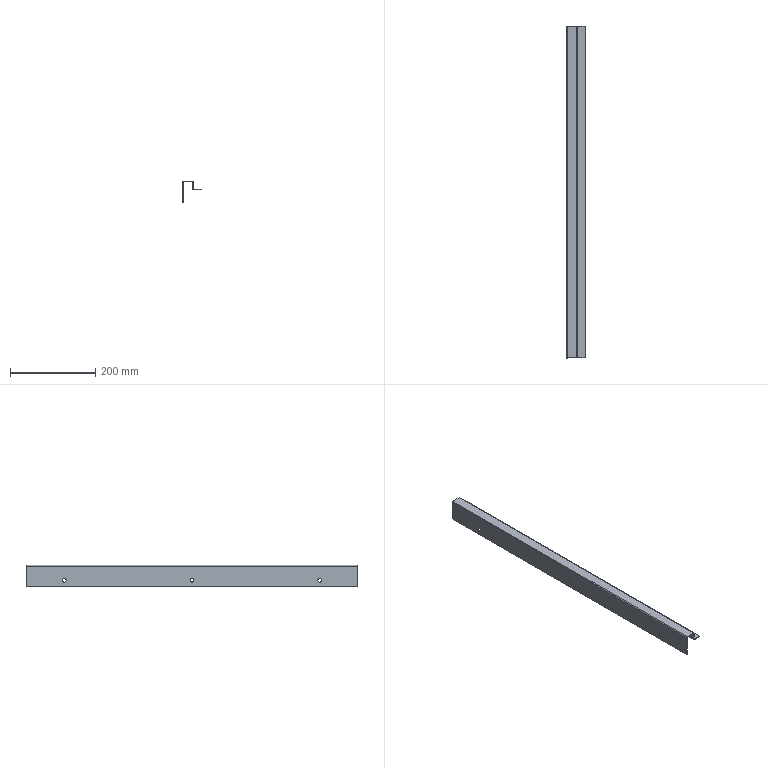Component | SolidWorks | Column-1 | 1 solid | 36 faces | box 43.5 x 780 x 50 mm | volume 127718 mm3 | plane 24 | cylinder 12 | commonest cylinder face diameters 9 x6 3.2 x3 0.2 x3
STEP:
#1=CARTESIAN_POINT('',(-13.498,9.896,34.139));
#2=VERTEX_POINT('',#1);
#3=CARTESIAN_POINT('',(-13.498,9.896,34.494));
#4=VERTEX_POINT('',#3);
#5=CARTESIAN_POINT('',(-13.498,9.896,34.316));
#6=DIRECTION('',(-1.,-0.,0.));
#7=DIRECTION('',(0.,0.,1.));
#8=AXIS2_PLACEMENT_3D('',#5,#6,#7);
#9=CIRCLE('',#8,0.1772);
#10=EDGE_CURVE('',#2,#4,#9,.T.);
#11=ORIENTED_EDGE('',*,*,#10,.T.);
#12=CARTESIAN_POINT('',(-13.439,9.896,34.494));
#13=VERTEX_POINT('',#12);
#14=CARTESIAN_POINT('',(-13.833,9.896,34.494));
#15=DIRECTION('',(1.,0.,-0.));
#16=VECTOR('',#15,39.37);
#17=LINE('',#14,#16);
#18=EDGE_CURVE('',#4,#13,#17,.T.);
#19=ORIENTED_EDGE('',*,*,#18,.T.);
#20=CARTESIAN_POINT('',(-13.439,9.896,34.139));
#21=VERTEX_POINT('',#20);
#22=CARTESIAN_POINT('',(-13.439,9.896,34.316));
#23=DIRECTION('',(1.,0.,-0.));
#24=DIRECTION('',(0.,0.,-1.));
#25=AXIS2_PLACEMENT_3D('',#22,#23,#24);
#26=CIRCLE('',#25,0.1772);
#27=EDGE_CURVE('',#13,#21,#26,.T.);
#28=ORIENTED_EDGE('',*,*,#27,.T.);
#29=CARTESIAN_POINT('',(-13.833,9.896,34.139));
#30=DIRECTION('',(1.,0.,-0.));
#31=VECTOR('',#30,39.37);
#32=LINE('',#29,#31);
#33=EDGE_CURVE('',#2,#21,#32,.T.);
#34=ORIENTED_EDGE('',*,*,#33,.F.);
#35=EDGE_LOOP('',(#11,#19,#28,#34));
#36=FACE_OUTER_BOUND('',#35,.T.);
#37=CARTESIAN_POINT('',(-13.833,9.896,34.316));
#38=DIRECTION('',(1.,0.,-0.));
#39=DIRECTION('',(0.,0.,-1.));
#40=AXIS2_PLACEMENT_3D('',#37,#38,#39);
#41=CYLINDRICAL_SURFACE('',#40,0.1772);
#42=ADVANCED_FACE('',(#36),#41,.F.);
#43=CARTESIAN_POINT('',(-13.498,-13.726,34.139));
#44=VERTEX_POINT('',#43);
#45=CARTESIAN_POINT('',(-13.498,-13.726,34.494));
#46=VERTEX_POINT('',#45);
#47=CARTESIAN_POINT('',(-13.498,-13.726,34.316));
#48=DIRECTION('',(-1.,-0.,0.));
#49=DIRECTION('',(0.,0.,1.));
#50=AXIS2_PLACEMENT_3D('',#47,#48,#49);
#51=CIRCLE('',#50,0.1772);
#52=EDGE_CURVE('',#44,#46,#51,.T.);
#53=ORIENTED_EDGE('',*,*,#52,.T.);
#54=CARTESIAN_POINT('',(-13.439,-13.726,34.494));
#55=VERTEX_POINT('',#54);
#56=CARTESIAN_POINT('',(-13.833,-13.726,34.494));
#57=DIRECTION('',(1.,0.,-0.));
#58=VECTOR('',#57,39.37);
#59=LINE('',#56,#58);
#60=EDGE_CURVE('',#46,#55,#59,.T.);
#61=ORIENTED_EDGE('',*,*,#60,.T.);
#62=CARTESIAN_POINT('',(-13.439,-13.726,34.139));
#63=VERTEX_POINT('',#62);
#64=CARTESIAN_POINT('',(-13.439,-13.726,34.316));
#65=DIRECTION('',(1.,0.,-0.));
#66=DIRECTION('',(0.,0.,-1.));
#67=AXIS2_PLACEMENT_3D('',#64,#65,#66);
#68=CIRCLE('',#67,0.1772);
#69=EDGE_CURVE('',#55,#63,#68,.T.);
#70=ORIENTED_EDGE('',*,*,#69,.T.);
#71=CARTESIAN_POINT('',(-13.833,-13.726,34.139));
#72=DIRECTION('',(1.,0.,-0.));
#73=VECTOR('',#72,39.37);
#74=LINE('',#71,#73);
#75=EDGE_CURVE('',#44,#63,#74,.T.);
#76=ORIENTED_EDGE('',*,*,#75,.F.);
#77=EDGE_LOOP('',(#53,#61,#70,#76));
#78=FACE_OUTER_BOUND('',#77,.T.);
#79=CARTESIAN_POINT('',(-13.833,-13.726,34.316));
#80=DIRECTION('',(1.,0.,-0.));
#81=DIRECTION('',(0.,0.,-1.));
#82=AXIS2_PLACEMENT_3D('',#79,#80,#81);
#83=CYLINDRICAL_SURFACE('',#82,0.1772);
#84=ADVANCED_FACE('',(#78),#83,.F.);
#85=CARTESIAN_POINT('',(-13.498,-1.915,34.139));
#86=VERTEX_POINT('',#85);
#87=CARTESIAN_POINT('',(-13.498,-1.915,34.494));
#88=VERTEX_POINT('',#87);
#89=CARTESIAN_POINT('',(-13.498,-1.915,34.316));
#90=DIRECTION('',(-1.,-0.,0.));
#91=DIRECTION('',(0.,0.,1.));
#92=AXIS2_PLACEMENT_3D('',#89,#90,#91);
#93=CIRCLE('',#92,0.1772);
#94=EDGE_CURVE('',#86,#88,#93,.T.);
#95=ORIENTED_EDGE('',*,*,#94,.T.);
#96=CARTESIAN_POINT('',(-13.439,-1.915,34.494));
#97=VERTEX_POINT('',#96);
#98=CARTESIAN_POINT('',(-13.833,-1.915,34.494));
#99=DIRECTION('',(1.,0.,-0.));
#100=VECTOR('',#99,39.37);
#101=LINE('',#98,#100);
#102=EDGE_CURVE('',#88,#97,#101,.T.);
#103=ORIENTED_EDGE('',*,*,#102,.T.);
#104=CARTESIAN_POINT('',(-13.439,-1.915,34.139));
#105=VERTEX_POINT('',#104);
#106=CARTESIAN_POINT('',(-13.439,-1.915,34.316));
#107=DIRECTION('',(1.,0.,-0.));
#108=DIRECTION('',(0.,0.,-1.));
#109=AXIS2_PLACEMENT_3D('',#106,#107,#108);
#110=CIRCLE('',#109,0.1772);
#111=EDGE_CURVE('',#97,#105,#110,.T.);
#112=ORIENTED_EDGE('',*,*,#111,.T.);
#113=CARTESIAN_POINT('',(-13.833,-1.915,34.139));
#114=DIRECTION('',(1.,0.,-0.));
#115=VECTOR('',#114,39.37);
#116=LINE('',#113,#115);
#117=EDGE_CURVE('',#86,#105,#116,.T.);
#118=ORIENTED_EDGE('',*,*,#117,.F.);
#119=EDGE_LOOP('',(#95,#103,#112,#118));
#120=FACE_OUTER_BOUND('',#119,.T.);
#121=CARTESIAN_POINT('',(-13.833,-1.915,34.316));
#122=DIRECTION('',(1.,0.,-0.));
#123=DIRECTION('',(0.,0.,-1.));
#124=AXIS2_PLACEMENT_3D('',#121,#122,#123);
#125=CYLINDRICAL_SURFACE('',#124,0.1772);
#126=ADVANCED_FACE('',(#120),#125,.F.);
#127=CARTESIAN_POINT('',(-12.514,13.44,35.631));
#128=VERTEX_POINT('',#127);
#129=CARTESIAN_POINT('',(-12.514,13.44,34.97));
#130=VERTEX_POINT('',#129);
#131=CARTESIAN_POINT('',(-12.514,13.44,34.907));
#132=DIRECTION('',(0.,0.,-1.));
#133=VECTOR('',#132,39.37);
#134=LINE('',#131,#133);
#135=EDGE_CURVE('',#128,#130,#134,.T.);
#136=ORIENTED_EDGE('',*,*,#135,.T.);
#137=CARTESIAN_POINT('',(-12.573,13.44,34.97));
#138=VERTEX_POINT('',#137);
#139=CARTESIAN_POINT('',(-12.514,13.44,34.97));
#140=DIRECTION('',(-1.,0.,0.));
#141=VECTOR('',#140,39.37);
#142=LINE('',#139,#141);
#143=EDGE_CURVE('',#130,#138,#142,.T.);
#144=ORIENTED_EDGE('',*,*,#143,.T.);
#145=CARTESIAN_POINT('',(-12.573,13.44,35.631));
#146=VERTEX_POINT('',#145);
#147=CARTESIAN_POINT('',(-12.573,13.44,35.694));
#148=DIRECTION('',(0.,0.,-1.));
#149=VECTOR('',#148,39.37);
#150=LINE('',#147,#149);
#151=EDGE_CURVE('',#146,#138,#150,.T.);
#152=ORIENTED_EDGE('',*,*,#151,.F.);
#153=CARTESIAN_POINT('',(-12.514,13.44,35.631));
#154=DIRECTION('',(1.,0.,0.));
#155=VECTOR('',#154,39.37);
#156=LINE('',#153,#155);
#157=EDGE_CURVE('',#146,#128,#156,.T.);
#158=ORIENTED_EDGE('',*,*,#157,.T.);
#159=EDGE_LOOP('',(#136,#144,#152,#158));
#160=FACE_OUTER_BOUND('',#159,.T.);
#161=CARTESIAN_POINT('',(-12.514,13.44,34.907));
#162=DIRECTION('',(-0.,1.,-0.));
#163=DIRECTION('',(-1.,-0.,0.));
#164=AXIS2_PLACEMENT_3D('',#161,#162,#163);
#165=PLANE('',#164);
#166=ADVANCED_FACE('',(#160),#165,.T.);
#167=CARTESIAN_POINT('',(-12.514,-17.269,34.97));
#168=VERTEX_POINT('',#167);
#169=CARTESIAN_POINT('',(-12.514,-17.269,35.631));
#170=VERTEX_POINT('',#169);
#171=CARTESIAN_POINT('',(-12.514,-17.269,35.635));
#172=DIRECTION('',(-0.,-0.,1.));
#173=VECTOR('',#172,39.37);
#174=LINE('',#171,#173);
#175=EDGE_CURVE('',#168,#170,#174,.T.);
#176=ORIENTED_EDGE('',*,*,#175,.F.);
#177=CARTESIAN_POINT('',(-12.514,13.44,34.97));
#178=DIRECTION('',(0.,-1.,0.));
#179=VECTOR('',#178,39.37);
#180=LINE('',#177,#179);
#181=EDGE_CURVE('',#130,#168,#180,.T.);
#182=ORIENTED_EDGE('',*,*,#181,.F.);
#183=ORIENTED_EDGE('',*,*,#135,.F.);
#184=CARTESIAN_POINT('',(-12.514,-1.915,35.631));
#185=DIRECTION('',(0.,-1.,0.));
#186=VECTOR('',#185,39.37);
#187=LINE('',#184,#186);
#188=EDGE_CURVE('',#128,#170,#187,.T.);
#189=ORIENTED_EDGE('',*,*,#188,.T.);
#190=EDGE_LOOP('',(#176,#182,#183,#189));
#191=FACE_OUTER_BOUND('',#190,.T.);
#192=CARTESIAN_POINT('',(-12.514,-1.915,35.694));
#193=DIRECTION('',(1.,0.,0.));
#194=DIRECTION('',(0.,0.,-1.));
#195=AXIS2_PLACEMENT_3D('',#192,#193,#194);
#196=PLANE('',#195);
#197=ADVANCED_FACE('',(#191),#196,.T.);
#198=CARTESIAN_POINT('',(-12.573,-17.269,34.97));
#199=VERTEX_POINT('',#198);
#200=CARTESIAN_POINT('',(-12.573,13.44,34.97));
#201=DIRECTION('',(0.,-1.,0.));
#202=VECTOR('',#201,39.37);
#203=LINE('',#200,#202);
#204=EDGE_CURVE('',#138,#199,#203,.T.);
#205=ORIENTED_EDGE('',*,*,#204,.T.);
#206=CARTESIAN_POINT('',(-12.573,-17.269,35.631));
#207=VERTEX_POINT('',#206);
#208=CARTESIAN_POINT('',(-12.573,-17.269,35.694));
#209=DIRECTION('',(-0.,-0.,1.));
#210=VECTOR('',#209,39.37);
#211=LINE('',#208,#210);
#212=EDGE_CURVE('',#199,#207,#211,.T.);
#213=ORIENTED_EDGE('',*,*,#212,.T.);
#214=CARTESIAN_POINT('',(-12.573,13.44,35.631));
#215=DIRECTION('',(0.,-1.,0.));
#216=VECTOR('',#215,39.37);
#217=LINE('',#214,#216);
#218=EDGE_CURVE('',#146,#207,#217,.T.);
#219=ORIENTED_EDGE('',*,*,#218,.F.);
#220=ORIENTED_EDGE('',*,*,#151,.T.);
#221=EDGE_LOOP('',(#205,#213,#219,#220));
#222=FACE_OUTER_BOUND('',#221,.T.);
#223=CARTESIAN_POINT('',(-12.573,-1.915,35.694));
#224=DIRECTION('',(1.,0.,0.));
#225=DIRECTION('',(0.,0.,-1.));
#226=AXIS2_PLACEMENT_3D('',#223,#224,#225);
#227=PLANE('',#226);
#228=ADVANCED_FACE('',(#222),#227,.F.);
#229=CARTESIAN_POINT('',(-12.577,-17.269,35.635));
#230=VERTEX_POINT('',#229);
#231=CARTESIAN_POINT('',(-12.577,13.44,35.635));
#232=VERTEX_POINT('',#231);
#233=CARTESIAN_POINT('',(-12.577,-17.269,35.635));
#234=DIRECTION('',(0.,1.,0.));
#235=VECTOR('',#234,39.37);
#236=LINE('',#233,#235);
#237=EDGE_CURVE('',#230,#232,#236,.T.);
#238=ORIENTED_EDGE('',*,*,#237,.F.);
#239=CARTESIAN_POINT('',(-13.435,-17.269,35.635));
#240=VERTEX_POINT('',#239);
#241=CARTESIAN_POINT('',(-13.498,-17.269,35.635));
#242=DIRECTION('',(1.,0.,0.));
#243=VECTOR('',#242,39.37);
#244=LINE('',#241,#243);
#245=EDGE_CURVE('',#240,#230,#244,.T.);
#246=ORIENTED_EDGE('',*,*,#245,.F.);
#247=CARTESIAN_POINT('',(-13.435,13.44,35.635));
#248=VERTEX_POINT('',#247);
#249=CARTESIAN_POINT('',(-13.435,13.44,35.635));
#250=DIRECTION('',(0.,-1.,0.));
#251=VECTOR('',#250,39.37);
#252=LINE('',#249,#251);
#253=EDGE_CURVE('',#248,#240,#252,.T.);
#254=ORIENTED_EDGE('',*,*,#253,.F.);
#255=CARTESIAN_POINT('',(-13.498,13.44,35.635));
#256=DIRECTION('',(-1.,0.,0.));
#257=VECTOR('',#256,39.37);
#258=LINE('',#255,#257);
#259=EDGE_CURVE('',#232,#248,#258,.T.);
#260=ORIENTED_EDGE('',*,*,#259,.F.);
#261=EDGE_LOOP('',(#238,#246,#254,#260));
#262=FACE_OUTER_BOUND('',#261,.T.);
#263=CARTESIAN_POINT('',(-13.006,-1.915,35.635));
#264=DIRECTION('',(0.,0.,1.));
#265=DIRECTION('',(1.,0.,0.));
#266=AXIS2_PLACEMENT_3D('',#263,#264,#265);
#267=PLANE('',#266);
#268=ADVANCED_FACE('',(#262),#267,.F.);
#269=CARTESIAN_POINT('',(-13.435,-17.269,35.694));
#270=VERTEX_POINT('',#269);
#271=CARTESIAN_POINT('',(-12.577,-17.269,35.694));
#272=VERTEX_POINT('',#271);
#273=CARTESIAN_POINT('',(-13.498,-17.269,35.694));
#274=DIRECTION('',(1.,0.,0.));
#275=VECTOR('',#274,39.37);
#276=LINE('',#273,#275);
#277=EDGE_CURVE('',#270,#272,#276,.T.);
#278=ORIENTED_EDGE('',*,*,#277,.T.);
#279=CARTESIAN_POINT('',(-12.577,13.44,35.694));
#280=VERTEX_POINT('',#279);
#281=CARTESIAN_POINT('',(-12.577,-17.269,35.694));
#282=DIRECTION('',(0.,1.,0.));
#283=VECTOR('',#282,39.37);
#284=LINE('',#281,#283);
#285=EDGE_CURVE('',#272,#280,#284,.T.);
#286=ORIENTED_EDGE('',*,*,#285,.T.);
#287=CARTESIAN_POINT('',(-13.435,13.44,35.694));
#288=VERTEX_POINT('',#287);
#289=CARTESIAN_POINT('',(-13.498,13.44,35.694));
#290=DIRECTION('',(-1.,0.,0.));
#291=VECTOR('',#290,39.37);
#292=LINE('',#289,#291);
#293=EDGE_CURVE('',#280,#288,#292,.T.);
#294=ORIENTED_EDGE('',*,*,#293,.T.);
#295=CARTESIAN_POINT('',(-13.435,13.44,35.694));
#296=DIRECTION('',(0.,-1.,0.));
#297=VECTOR('',#296,39.37);
#298=LINE('',#295,#297);
#299=EDGE_CURVE('',#288,#270,#298,.T.);
#300=ORIENTED_EDGE('',*,*,#299,.T.);
#301=EDGE_LOOP('',(#278,#286,#294,#300));
#302=FACE_OUTER_BOUND('',#301,.T.);
#303=CARTESIAN_POINT('',(-13.006,-1.915,35.694));
#304=DIRECTION('',(0.,0.,1.));
#305=DIRECTION('',(1.,0.,0.));
#306=AXIS2_PLACEMENT_3D('',#303,#304,#305);
#307=PLANE('',#306);
#308=ADVANCED_FACE('',(#302),#307,.T.);
#309=ORIENTED_EDGE('',*,*,#245,.T.);
#310=CARTESIAN_POINT('',(-12.577,-17.269,35.635));
#311=DIRECTION('',(0.,0.,1.));
#312=VECTOR('',#311,39.37);
#313=LINE('',#310,#312);
#314=EDGE_CURVE('',#230,#272,#313,.T.);
#315=ORIENTED_EDGE('',*,*,#314,.T.);
#316=ORIENTED_EDGE('',*,*,#277,.F.);
#317=CARTESIAN_POINT('',(-13.435,-17.269,35.635));
#318=DIRECTION('',(-0.,0.,1.));
#319=VECTOR('',#318,39.37);
#320=LINE('',#317,#319);
#321=EDGE_CURVE('',#240,#270,#320,.T.);
#322=ORIENTED_EDGE('',*,*,#321,.F.);
#323=EDGE_LOOP('',(#309,#315,#316,#322));
#324=FACE_OUTER_BOUND('',#323,.T.);
#325=CARTESIAN_POINT('',(-13.498,-17.269,35.635));
#326=DIRECTION('',(0.,-1.,0.));
#327=DIRECTION('',(0.,0.,-1.));
#328=AXIS2_PLACEMENT_3D('',#325,#326,#327);
#329=PLANE('',#328);
#330=ADVANCED_FACE('',(#324),#329,.T.);
#331=CARTESIAN_POINT('',(-12.577,13.44,35.635));
#332=DIRECTION('',(0.,0.,1.));
#333=VECTOR('',#332,39.37);
#334=LINE('',#331,#333);
#335=EDGE_CURVE('',#232,#280,#334,.T.);
#336=ORIENTED_EDGE('',*,*,#335,.F.);
#337=ORIENTED_EDGE('',*,*,#259,.T.);
#338=CARTESIAN_POINT('',(-13.435,13.44,35.635));
#339=DIRECTION('',(-0.,0.,1.));
#340=VECTOR('',#339,39.37);
#341=LINE('',#338,#340);
#342=EDGE_CURVE('',#248,#288,#341,.T.);
#343=ORIENTED_EDGE('',*,*,#342,.T.);
#344=ORIENTED_EDGE('',*,*,#293,.F.);
#345=EDGE_LOOP('',(#336,#337,#343,#344));
#346=FACE_OUTER_BOUND('',#345,.T.);
#347=CARTESIAN_POINT('',(-13.498,13.44,35.635));
#348=DIRECTION('',(0.,1.,0.));
#349=DIRECTION('',(0.,0.,1.));
#350=AXIS2_PLACEMENT_3D('',#347,#348,#349);
#351=PLANE('',#350);
#352=ADVANCED_FACE('',(#346),#351,.T.);
#353=CARTESIAN_POINT('',(-13.439,-17.269,35.631));
#354=VERTEX_POINT('',#353);
#355=CARTESIAN_POINT('',(-13.498,-17.269,35.631));
#356=VERTEX_POINT('',#355);
#357=CARTESIAN_POINT('',(-13.498,-17.269,35.631));
#358=DIRECTION('',(-1.,-0.,0.));
#359=VECTOR('',#358,39.37);
#360=LINE('',#357,#359);
#361=EDGE_CURVE('',#354,#356,#360,.T.);
#362=ORIENTED_EDGE('',*,*,#361,.F.);
#363=CARTESIAN_POINT('',(-13.435,-17.269,35.631));
#364=DIRECTION('',(0.,-1.,0.));
#365=DIRECTION('',(-0.,0.,1.));
#366=AXIS2_PLACEMENT_3D('',#363,#364,#365);
#367=CIRCLE('',#366,0.003937);
#368=EDGE_CURVE('',#240,#354,#367,.T.);
#369=ORIENTED_EDGE('',*,*,#368,.F.);
#370=ORIENTED_EDGE('',*,*,#321,.T.);
#371=CARTESIAN_POINT('',(-13.435,-17.269,35.631));
#372=DIRECTION('',(0.,-1.,0.));
#373=DIRECTION('',(-0.,0.,1.));
#374=AXIS2_PLACEMENT_3D('',#371,#372,#373);
#375=CIRCLE('',#374,0.06299);
#376=EDGE_CURVE('',#270,#356,#375,.T.);
#377=ORIENTED_EDGE('',*,*,#376,.T.);
#378=EDGE_LOOP('',(#362,#369,#370,#377));
#379=FACE_OUTER_BOUND('',#378,.T.);
#380=CARTESIAN_POINT('',(-13.435,-17.269,35.631));
#381=DIRECTION('',(0.,-1.,0.));
#382=DIRECTION('',(0.,0.,-1.));
#383=AXIS2_PLACEMENT_3D('',#380,#381,#382);
#384=PLANE('',#383);
#385=ADVANCED_FACE('',(#379),#384,.T.);
#386=CARTESIAN_POINT('',(-13.439,13.44,35.631));
#387=VERTEX_POINT('',#386);
#388=CARTESIAN_POINT('',(-13.435,13.44,35.631));
#389=DIRECTION('',(0.,1.,0.));
#390=DIRECTION('',(0.,0.,1.));
#391=AXIS2_PLACEMENT_3D('',#388,#389,#390);
#392=CIRCLE('',#391,0.003937);
#393=EDGE_CURVE('',#387,#248,#392,.T.);
#394=ORIENTED_EDGE('',*,*,#393,.F.);
#395=CARTESIAN_POINT('',(-13.498,13.44,35.631));
#396=VERTEX_POINT('',#395);
#397=CARTESIAN_POINT('',(-13.439,13.44,35.631));
#398=DIRECTION('',(-1.,-0.,0.));
#399=VECTOR('',#398,39.37);
#400=LINE('',#397,#399);
#401=EDGE_CURVE('',#387,#396,#400,.T.);
#402=ORIENTED_EDGE('',*,*,#401,.T.);
#403=CARTESIAN_POINT('',(-13.435,13.44,35.631));
#404=DIRECTION('',(0.,1.,0.));
#405=DIRECTION('',(0.,0.,1.));
#406=AXIS2_PLACEMENT_3D('',#403,#404,#405);
#407=CIRCLE('',#406,0.06299);
#408=EDGE_CURVE('',#396,#288,#407,.T.);
#409=ORIENTED_EDGE('',*,*,#408,.T.);
#410=ORIENTED_EDGE('',*,*,#342,.F.);
#411=EDGE_LOOP('',(#394,#402,#409,#410));
#412=FACE_OUTER_BOUND('',#411,.T.);
#413=CARTESIAN_POINT('',(-13.435,13.44,35.631));
#414=DIRECTION('',(0.,-1.,0.));
#415=DIRECTION('',(0.,0.,-1.));
#416=AXIS2_PLACEMENT_3D('',#413,#414,#415);
#417=PLANE('',#416);
#418=ADVANCED_FACE('',(#412),#417,.F.);
#419=ORIENTED_EDGE('',*,*,#299,.F.);
#420=ORIENTED_EDGE('',*,*,#408,.F.);
#421=CARTESIAN_POINT('',(-13.498,-1.915,35.631));
#422=DIRECTION('',(-0.,1.,0.));
#423=VECTOR('',#422,39.37);
#424=LINE('',#421,#423);
#425=EDGE_CURVE('',#356,#396,#424,.T.);
#426=ORIENTED_EDGE('',*,*,#425,.F.);
#427=ORIENTED_EDGE('',*,*,#376,.F.);
#428=EDGE_LOOP('',(#419,#420,#426,#427));
#429=FACE_OUTER_BOUND('',#428,.T.);
#430=CARTESIAN_POINT('',(-13.435,13.44,35.631));
#431=DIRECTION('',(0.,1.,0.));
#432=DIRECTION('',(-1.,0.,0.));
#433=AXIS2_PLACEMENT_3D('',#430,#431,#432);
#434=CYLINDRICAL_SURFACE('',#433,0.06299);
#435=ADVANCED_FACE('',(#429),#434,.T.);
#436=ORIENTED_EDGE('',*,*,#253,.T.);
#437=ORIENTED_EDGE('',*,*,#368,.T.);
#438=CARTESIAN_POINT('',(-13.439,-17.269,35.631));
#439=DIRECTION('',(-0.,1.,0.));
#440=VECTOR('',#439,39.37);
#441=LINE('',#438,#440);
#442=EDGE_CURVE('',#354,#387,#441,.T.);
#443=ORIENTED_EDGE('',*,*,#442,.T.);
#444=ORIENTED_EDGE('',*,*,#393,.T.);
#445=EDGE_LOOP('',(#436,#437,#443,#444));
#446=FACE_OUTER_BOUND('',#445,.T.);
#447=CARTESIAN_POINT('',(-13.435,13.44,35.631));
#448=DIRECTION('',(0.,1.,0.));
#449=DIRECTION('',(-1.,0.,0.));
#450=AXIS2_PLACEMENT_3D('',#447,#448,#449);
#451=CYLINDRICAL_SURFACE('',#450,0.003937);
#452=ADVANCED_FACE('',(#446),#451,.F.);
#453=CARTESIAN_POINT('',(-13.498,13.44,33.726));
#454=VERTEX_POINT('',#453);
#455=CARTESIAN_POINT('',(-13.498,13.44,35.635));
#456=DIRECTION('',(0.,0.,1.));
#457=VECTOR('',#456,39.37);
#458=LINE('',#455,#457);
#459=EDGE_CURVE('',#454,#396,#458,.T.);
#460=ORIENTED_EDGE('',*,*,#459,.T.);
#461=ORIENTED_EDGE('',*,*,#401,.F.);
#462=CARTESIAN_POINT('',(-13.439,13.44,33.726));
#463=VERTEX_POINT('',#462);
#464=CARTESIAN_POINT('',(-13.439,13.44,35.694));
#465=DIRECTION('',(0.,0.,1.));
#466=VECTOR('',#465,39.37);
#467=LINE('',#464,#466);
#468=EDGE_CURVE('',#463,#387,#467,.T.);
#469=ORIENTED_EDGE('',*,*,#468,.F.);
#470=CARTESIAN_POINT('',(-13.498,13.44,33.726));
#471=DIRECTION('',(1.,0.,-0.));
#472=VECTOR('',#471,39.37);
#473=LINE('',#470,#472);
#474=EDGE_CURVE('',#454,#463,#473,.T.);
#475=ORIENTED_EDGE('',*,*,#474,.F.);
#476=EDGE_LOOP('',(#460,#461,#469,#475));
#477=FACE_OUTER_BOUND('',#476,.T.);
#478=CARTESIAN_POINT('',(-13.498,13.44,35.635));
#479=DIRECTION('',(-0.,1.,0.));
#480=DIRECTION('',(-1.,-0.,0.));
#481=AXIS2_PLACEMENT_3D('',#478,#479,#480);
#482=PLANE('',#481);
#483=ADVANCED_FACE('',(#477),#482,.T.);
#484=CARTESIAN_POINT('',(-13.439,-17.269,33.726));
#485=VERTEX_POINT('',#484);
#486=CARTESIAN_POINT('',(-13.439,-17.269,35.694));
#487=DIRECTION('',(-0.,0.,-1.));
#488=VECTOR('',#487,39.37);
#489=LINE('',#486,#488);
#490=EDGE_CURVE('',#354,#485,#489,.T.);
#491=ORIENTED_EDGE('',*,*,#490,.F.);
#492=ORIENTED_EDGE('',*,*,#361,.T.);
#493=CARTESIAN_POINT('',(-13.498,-17.269,33.726));
#494=VERTEX_POINT('',#493);
#495=CARTESIAN_POINT('',(-13.498,-17.269,33.726));
#496=DIRECTION('',(-0.,0.,-1.));
#497=VECTOR('',#496,39.37);
#498=LINE('',#495,#497);
#499=EDGE_CURVE('',#356,#494,#498,.T.);
#500=ORIENTED_EDGE('',*,*,#499,.T.);
#501=CARTESIAN_POINT('',(-13.498,-17.269,33.726));
#502=DIRECTION('',(1.,0.,-0.));
#503=VECTOR('',#502,39.37);
#504=LINE('',#501,#503);
#505=EDGE_CURVE('',#494,#485,#504,.T.);
#506=ORIENTED_EDGE('',*,*,#505,.T.);
#507=EDGE_LOOP('',(#491,#492,#500,#506));
#508=FACE_OUTER_BOUND('',#507,.T.);
#509=CARTESIAN_POINT('',(-13.498,-17.269,33.726));
#510=DIRECTION('',(0.,-1.,-0.));
#511=DIRECTION('',(1.,0.,0.));
#512=AXIS2_PLACEMENT_3D('',#509,#510,#511);
#513=PLANE('',#512);
#514=ADVANCED_FACE('',(#508),#513,.T.);
#515=ORIENTED_EDGE('',*,*,#52,.F.);
#516=CARTESIAN_POINT('',(-13.498,-13.726,34.316));
#517=DIRECTION('',(-1.,-0.,0.));
#518=DIRECTION('',(0.,0.,1.));
#519=AXIS2_PLACEMENT_3D('',#516,#517,#518);
#520=CIRCLE('',#519,0.1772);
#521=EDGE_CURVE('',#46,#44,#520,.T.);
#522=ORIENTED_EDGE('',*,*,#521,.F.);
#523=EDGE_LOOP('',(#515,#522));
#524=FACE_BOUND('',#523,.T.);
#525=ORIENTED_EDGE('',*,*,#94,.F.);
#526=CARTESIAN_POINT('',(-13.498,-1.915,34.316));
#527=DIRECTION('',(-1.,-0.,0.));
#528=DIRECTION('',(0.,0.,1.));
#529=AXIS2_PLACEMENT_3D('',#526,#527,#528);
#530=CIRCLE('',#529,0.1772);
#531=EDGE_CURVE('',#88,#86,#530,.T.);
#532=ORIENTED_EDGE('',*,*,#531,.F.);
#533=EDGE_LOOP('',(#525,#532));
#534=FACE_BOUND('',#533,.T.);
#535=ORIENTED_EDGE('',*,*,#499,.F.);
#536=ORIENTED_EDGE('',*,*,#425,.T.);
#537=ORIENTED_EDGE('',*,*,#459,.F.);
#538=CARTESIAN_POINT('',(-13.498,13.44,33.726));
#539=DIRECTION('',(-0.,1.,0.));
#540=VECTOR('',#539,39.37);
#541=LINE('',#538,#540);
#542=EDGE_CURVE('',#494,#454,#541,.T.);
#543=ORIENTED_EDGE('',*,*,#542,.F.);
#544=EDGE_LOOP('',(#535,#536,#537,#543));
#545=FACE_OUTER_BOUND('',#544,.T.);
#546=ORIENTED_EDGE('',*,*,#10,.F.);
#547=CARTESIAN_POINT('',(-13.498,9.896,34.316));
#548=DIRECTION('',(-1.,-0.,0.));
#549=DIRECTION('',(0.,0.,1.));
#550=AXIS2_PLACEMENT_3D('',#547,#548,#549);
#551=CIRCLE('',#550,0.1772);
#552=EDGE_CURVE('',#4,#2,#551,.T.);
#553=ORIENTED_EDGE('',*,*,#552,.F.);
#554=EDGE_LOOP('',(#546,#553));
#555=FACE_BOUND('',#554,.T.);
#556=CARTESIAN_POINT('',(-13.498,-1.915,35.694));
#557=DIRECTION('',(-1.,-0.,0.));
#558=DIRECTION('',(0.,0.,1.));
#559=AXIS2_PLACEMENT_3D('',#556,#557,#558);
#560=PLANE('',#559);
#561=ADVANCED_FACE('',(#524,#534,#545,#555),#560,.T.);
#562=CARTESIAN_POINT('',(-13.439,-13.726,34.316));
#563=DIRECTION('',(1.,0.,-0.));
#564=DIRECTION('',(0.,0.,-1.));
#565=AXIS2_PLACEMENT_3D('',#562,#563,#564);
#566=CIRCLE('',#565,0.1772);
#567=EDGE_CURVE('',#63,#55,#566,.T.);
#568=ORIENTED_EDGE('',*,*,#567,.F.);
#569=ORIENTED_EDGE('',*,*,#69,.F.);
#570=EDGE_LOOP('',(#568,#569));
#571=FACE_BOUND('',#570,.T.);
#572=CARTESIAN_POINT('',(-13.439,-1.915,34.316));
#573=DIRECTION('',(1.,0.,-0.));
#574=DIRECTION('',(0.,0.,-1.));
#575=AXIS2_PLACEMENT_3D('',#572,#573,#574);
#576=CIRCLE('',#575,0.1772);
#577=EDGE_CURVE('',#105,#97,#576,.T.);
#578=ORIENTED_EDGE('',*,*,#577,.F.);
#579=ORIENTED_EDGE('',*,*,#111,.F.);
#580=EDGE_LOOP('',(#578,#579));
#581=FACE_BOUND('',#580,.T.);
#582=ORIENTED_EDGE('',*,*,#442,.F.);
#583=ORIENTED_EDGE('',*,*,#490,.T.);
#584=CARTESIAN_POINT('',(-13.439,-1.915,33.726));
#585=DIRECTION('',(-0.,1.,0.));
#586=VECTOR('',#585,39.37);
#587=LINE('',#584,#586);
#588=EDGE_CURVE('',#485,#463,#587,.T.);
#589=ORIENTED_EDGE('',*,*,#588,.T.);
#590=ORIENTED_EDGE('',*,*,#468,.T.);
#591=EDGE_LOOP('',(#582,#583,#589,#590));
#592=FACE_OUTER_BOUND('',#591,.T.);
#593=CARTESIAN_POINT('',(-13.439,9.896,34.316));
#594=DIRECTION('',(1.,0.,-0.));
#595=DIRECTION('',(0.,0.,-1.));
#596=AXIS2_PLACEMENT_3D('',#593,#594,#595);
#597=CIRCLE('',#596,0.1772);
#598=EDGE_CURVE('',#21,#13,#597,.T.);
#599=ORIENTED_EDGE('',*,*,#598,.F.);
#600=ORIENTED_EDGE('',*,*,#27,.F.);
#601=EDGE_LOOP('',(#599,#600));
#602=FACE_BOUND('',#601,.T.);
#603=CARTESIAN_POINT('',(-13.439,-1.915,35.694));
#604=DIRECTION('',(-1.,-0.,0.));
#605=DIRECTION('',(0.,0.,1.));
#606=AXIS2_PLACEMENT_3D('',#603,#604,#605);
#607=PLANE('',#606);
#608=ADVANCED_FACE('',(#571,#581,#592,#602),#607,.F.);
#609=ORIENTED_EDGE('',*,*,#588,.F.);
#610=ORIENTED_EDGE('',*,*,#505,.F.);
#611=ORIENTED_EDGE('',*,*,#542,.T.);
#612=ORIENTED_EDGE('',*,*,#474,.T.);
#613=EDGE_LOOP('',(#609,#610,#611,#612));
#614=FACE_OUTER_BOUND('',#613,.T.);
#615=CARTESIAN_POINT('',(-13.498,13.44,33.726));
#616=DIRECTION('',(-0.,-0.,-1.));
#617=DIRECTION('',(-1.,0.,0.));
#618=AXIS2_PLACEMENT_3D('',#615,#616,#617);
#619=PLANE('',#618);
#620=ADVANCED_FACE('',(#614),#619,.T.);
#621=ORIENTED_EDGE('',*,*,#157,.F.);
#622=CARTESIAN_POINT('',(-12.577,13.44,35.631));
#623=DIRECTION('',(0.,1.,0.));
#624=DIRECTION('',(0.,0.,-1.));
#625=AXIS2_PLACEMENT_3D('',#622,#623,#624);
#626=CIRCLE('',#625,0.003937);
#627=EDGE_CURVE('',#232,#146,#626,.T.);
#628=ORIENTED_EDGE('',*,*,#627,.F.);
#629=ORIENTED_EDGE('',*,*,#335,.T.);
#630=CARTESIAN_POINT('',(-12.577,13.44,35.631));
#631=DIRECTION('',(0.,1.,0.));
#632=DIRECTION('',(0.,0.,-1.));
#633=AXIS2_PLACEMENT_3D('',#630,#631,#632);
#634=CIRCLE('',#633,0.06299);
#635=EDGE_CURVE('',#280,#128,#634,.T.);
#636=ORIENTED_EDGE('',*,*,#635,.T.);
#637=EDGE_LOOP('',(#621,#628,#629,#636));
#638=FACE_OUTER_BOUND('',#637,.T.);
#639=CARTESIAN_POINT('',(-12.577,13.44,35.631));
#640=DIRECTION('',(0.,1.,0.));
#641=DIRECTION('',(0.,0.,1.));
#642=AXIS2_PLACEMENT_3D('',#639,#640,#641);
#643=PLANE('',#642);
#644=ADVANCED_FACE('',(#638),#643,.T.);
#645=CARTESIAN_POINT('',(-12.577,-17.269,35.631));
#646=DIRECTION('',(0.,-1.,0.));
#647=DIRECTION('',(0.,0.,-1.));
#648=AXIS2_PLACEMENT_3D('',#645,#646,#647);
#649=CIRCLE('',#648,0.003937);
#650=EDGE_CURVE('',#207,#230,#649,.T.);
#651=ORIENTED_EDGE('',*,*,#650,.F.);
#652=CARTESIAN_POINT('',(-12.573,-17.269,35.631));
#653=DIRECTION('',(1.,0.,0.));
#654=VECTOR('',#653,39.37);
#655=LINE('',#652,#654);
#656=EDGE_CURVE('',#207,#170,#655,.T.);
#657=ORIENTED_EDGE('',*,*,#656,.T.);
#658=CARTESIAN_POINT('',(-12.577,-17.269,35.631));
#659=DIRECTION('',(0.,-1.,0.));
#660=DIRECTION('',(0.,0.,-1.));
#661=AXIS2_PLACEMENT_3D('',#658,#659,#660);
#662=CIRCLE('',#661,0.06299);
#663=EDGE_CURVE('',#170,#272,#662,.T.);
#664=ORIENTED_EDGE('',*,*,#663,.T.);
#665=ORIENTED_EDGE('',*,*,#314,.F.);
#666=EDGE_LOOP('',(#651,#657,#664,#665));
#667=FACE_OUTER_BOUND('',#666,.T.);
#668=CARTESIAN_POINT('',(-12.577,-17.269,35.631));
#669=DIRECTION('',(0.,1.,0.));
#670=DIRECTION('',(0.,0.,1.));
#671=AXIS2_PLACEMENT_3D('',#668,#669,#670);
#672=PLANE('',#671);
#673=ADVANCED_FACE('',(#667),#672,.F.);
#674=ORIENTED_EDGE('',*,*,#285,.F.);
#675=ORIENTED_EDGE('',*,*,#663,.F.);
#676=ORIENTED_EDGE('',*,*,#188,.F.);
#677=ORIENTED_EDGE('',*,*,#635,.F.);
#678=EDGE_LOOP('',(#674,#675,#676,#677));
#679=FACE_OUTER_BOUND('',#678,.T.);
#680=CARTESIAN_POINT('',(-12.577,-17.269,35.631));
#681=DIRECTION('',(0.,-1.,0.));
#682=DIRECTION('',(1.,0.,0.));
#683=AXIS2_PLACEMENT_3D('',#680,#681,#682);
#684=CYLINDRICAL_SURFACE('',#683,0.06299);
#685=ADVANCED_FACE('',(#679),#684,.T.);
#686=ORIENTED_EDGE('',*,*,#237,.T.);
#687=ORIENTED_EDGE('',*,*,#627,.T.);
#688=ORIENTED_EDGE('',*,*,#218,.T.);
#689=ORIENTED_EDGE('',*,*,#650,.T.);
#690=EDGE_LOOP('',(#686,#687,#688,#689));
#691=FACE_OUTER_BOUND('',#690,.T.);
#692=CARTESIAN_POINT('',(-12.577,-17.269,35.631));
#693=DIRECTION('',(0.,-1.,0.));
#694=DIRECTION('',(1.,0.,0.));
#695=AXIS2_PLACEMENT_3D('',#692,#693,#694);
#696=CYLINDRICAL_SURFACE('',#695,0.003937);
#697=ADVANCED_FACE('',(#691),#696,.F.);
#698=CARTESIAN_POINT('',(-12.514,-17.269,34.97));
#699=DIRECTION('',(-1.,0.,0.));
#700=VECTOR('',#699,39.37);
#701=LINE('',#698,#700);
#702=EDGE_CURVE('',#168,#199,#701,.T.);
#703=ORIENTED_EDGE('',*,*,#702,.F.);
#704=ORIENTED_EDGE('',*,*,#175,.T.);
#705=ORIENTED_EDGE('',*,*,#656,.F.);
#706=ORIENTED_EDGE('',*,*,#212,.F.);
#707=EDGE_LOOP('',(#703,#704,#705,#706));
#708=FACE_OUTER_BOUND('',#707,.T.);
#709=CARTESIAN_POINT('',(-12.514,-17.269,35.635));
#710=DIRECTION('',(0.,-1.,0.));
#711=DIRECTION('',(1.,0.,0.));
#712=AXIS2_PLACEMENT_3D('',#709,#710,#711);
#713=PLANE('',#712);
#714=ADVANCED_FACE('',(#708),#713,.T.);
#715=CARTESIAN_POINT('',(-12.51,-17.269,34.966));
#716=VERTEX_POINT('',#715);
#717=CARTESIAN_POINT('',(-12.51,-17.269,34.907));
#718=VERTEX_POINT('',#717);
#719=CARTESIAN_POINT('',(-12.51,-17.269,34.907));
#720=DIRECTION('',(0.,0.,-1.));
#721=VECTOR('',#720,39.37);
#722=LINE('',#719,#721);
#723=EDGE_CURVE('',#716,#718,#722,.T.);
#724=ORIENTED_EDGE('',*,*,#723,.F.);
#725=CARTESIAN_POINT('',(-12.51,-17.269,34.97));
#726=DIRECTION('',(0.,-1.,0.));
#727=DIRECTION('',(0.,0.,1.));
#728=AXIS2_PLACEMENT_3D('',#725,#726,#727);
#729=CIRCLE('',#728,0.003937);
#730=EDGE_CURVE('',#168,#716,#729,.T.);
#731=ORIENTED_EDGE('',*,*,#730,.F.);
#732=ORIENTED_EDGE('',*,*,#702,.T.);
#733=CARTESIAN_POINT('',(-12.51,-17.269,34.97));
#734=DIRECTION('',(0.,-1.,0.));
#735=DIRECTION('',(0.,0.,1.));
#736=AXIS2_PLACEMENT_3D('',#733,#734,#735);
#737=CIRCLE('',#736,0.06299);
#738=EDGE_CURVE('',#199,#718,#737,.T.);
#739=ORIENTED_EDGE('',*,*,#738,.T.);
#740=EDGE_LOOP('',(#724,#731,#732,#739));
#741=FACE_OUTER_BOUND('',#740,.T.);
#742=CARTESIAN_POINT('',(-12.51,-17.269,34.97));
#743=DIRECTION('',(0.,-1.,0.));
#744=DIRECTION('',(0.,0.,-1.));
#745=AXIS2_PLACEMENT_3D('',#742,#743,#744);
#746=PLANE('',#745);
#747=ADVANCED_FACE('',(#741),#746,.T.);
#748=CARTESIAN_POINT('',(-12.51,13.44,34.966));
#749=VERTEX_POINT('',#748);
#750=CARTESIAN_POINT('',(-12.51,13.44,34.97));
#751=DIRECTION('',(0.,1.,0.));
#752=DIRECTION('',(0.,0.,1.));
#753=AXIS2_PLACEMENT_3D('',#750,#751,#752);
#754=CIRCLE('',#753,0.003937);
#755=EDGE_CURVE('',#749,#130,#754,.T.);
#756=ORIENTED_EDGE('',*,*,#755,.F.);
#757=CARTESIAN_POINT('',(-12.51,13.44,34.907));
#758=VERTEX_POINT('',#757);
#759=CARTESIAN_POINT('',(-12.51,13.44,34.966));
#760=DIRECTION('',(0.,0.,-1.));
#761=VECTOR('',#760,39.37);
#762=LINE('',#759,#761);
#763=EDGE_CURVE('',#749,#758,#762,.T.);
#764=ORIENTED_EDGE('',*,*,#763,.T.);
#765=CARTESIAN_POINT('',(-12.51,13.44,34.97));
#766=DIRECTION('',(0.,1.,0.));
#767=DIRECTION('',(0.,0.,1.));
#768=AXIS2_PLACEMENT_3D('',#765,#766,#767);
#769=CIRCLE('',#768,0.06299);
#770=EDGE_CURVE('',#758,#138,#769,.T.);
#771=ORIENTED_EDGE('',*,*,#770,.T.);
#772=ORIENTED_EDGE('',*,*,#143,.F.);
#773=EDGE_LOOP('',(#756,#764,#771,#772));
#774=FACE_OUTER_BOUND('',#773,.T.);
#775=CARTESIAN_POINT('',(-12.51,13.44,34.97));
#776=DIRECTION('',(0.,-1.,0.));
#777=DIRECTION('',(0.,0.,-1.));
#778=AXIS2_PLACEMENT_3D('',#775,#776,#777);
#779=PLANE('',#778);
#780=ADVANCED_FACE('',(#774),#779,.F.);
#781=ORIENTED_EDGE('',*,*,#204,.F.);
#782=ORIENTED_EDGE('',*,*,#770,.F.);
#783=CARTESIAN_POINT('',(-12.51,-1.915,34.907));
#784=DIRECTION('',(-0.,1.,0.));
#785=VECTOR('',#784,39.37);
#786=LINE('',#783,#785);
#787=EDGE_CURVE('',#718,#758,#786,.T.);
#788=ORIENTED_EDGE('',*,*,#787,.F.);
#789=ORIENTED_EDGE('',*,*,#738,.F.);
#790=EDGE_LOOP('',(#781,#782,#788,#789));
#791=FACE_OUTER_BOUND('',#790,.T.);
#792=CARTESIAN_POINT('',(-12.51,13.44,34.97));
#793=DIRECTION('',(0.,1.,0.));
#794=DIRECTION('',(0.,0.,-1.));
#795=AXIS2_PLACEMENT_3D('',#792,#793,#794);
#796=CYLINDRICAL_SURFACE('',#795,0.06299);
#797=ADVANCED_FACE('',(#791),#796,.T.);
#798=ORIENTED_EDGE('',*,*,#181,.T.);
#799=ORIENTED_EDGE('',*,*,#730,.T.);
#800=CARTESIAN_POINT('',(-12.51,-17.269,34.966));
#801=DIRECTION('',(-0.,1.,0.));
#802=VECTOR('',#801,39.37);
#803=LINE('',#800,#802);
#804=EDGE_CURVE('',#716,#749,#803,.T.);
#805=ORIENTED_EDGE('',*,*,#804,.T.);
#806=ORIENTED_EDGE('',*,*,#755,.T.);
#807=EDGE_LOOP('',(#798,#799,#805,#806));
#808=FACE_OUTER_BOUND('',#807,.T.);
#809=CARTESIAN_POINT('',(-12.51,13.44,34.97));
#810=DIRECTION('',(0.,1.,0.));
#811=DIRECTION('',(0.,0.,-1.));
#812=AXIS2_PLACEMENT_3D('',#809,#810,#811);
#813=CYLINDRICAL_SURFACE('',#812,0.003937);
#814=ADVANCED_FACE('',(#808),#813,.F.);
#815=CARTESIAN_POINT('',(-11.786,13.44,34.907));
#816=VERTEX_POINT('',#815);
#817=CARTESIAN_POINT('',(-12.514,13.44,34.907));
#818=DIRECTION('',(-1.,0.,0.));
#819=VECTOR('',#818,39.37);
#820=LINE('',#817,#819);
#821=EDGE_CURVE('',#816,#758,#820,.T.);
#822=ORIENTED_EDGE('',*,*,#821,.T.);
#823=ORIENTED_EDGE('',*,*,#763,.F.);
#824=CARTESIAN_POINT('',(-11.786,13.44,34.966));
#825=VERTEX_POINT('',#824);
#826=CARTESIAN_POINT('',(-13.006,13.44,34.966));
#827=DIRECTION('',(-1.,0.,0.));
#828=VECTOR('',#827,39.37);
#829=LINE('',#826,#828);
#830=EDGE_CURVE('',#825,#749,#829,.T.);
#831=ORIENTED_EDGE('',*,*,#830,.F.);
#832=CARTESIAN_POINT('',(-11.786,13.44,34.907));
#833=DIRECTION('',(-0.,-0.,1.));
#834=VECTOR('',#833,39.37);
#835=LINE('',#832,#834);
#836=EDGE_CURVE('',#816,#825,#835,.T.);
#837=ORIENTED_EDGE('',*,*,#836,.F.);
#838=EDGE_LOOP('',(#822,#823,#831,#837));
#839=FACE_OUTER_BOUND('',#838,.T.);
#840=CARTESIAN_POINT('',(-12.514,13.44,34.907));
#841=DIRECTION('',(0.,1.,0.));
#842=DIRECTION('',(0.,-0.,1.));
#843=AXIS2_PLACEMENT_3D('',#840,#841,#842);
#844=PLANE('',#843);
#845=ADVANCED_FACE('',(#839),#844,.T.);
#846=CARTESIAN_POINT('',(-11.786,-17.269,34.966));
#847=VERTEX_POINT('',#846);
#848=CARTESIAN_POINT('',(-13.006,-17.269,34.966));
#849=DIRECTION('',(1.,0.,0.));
#850=VECTOR('',#849,39.37);
#851=LINE('',#848,#850);
#852=EDGE_CURVE('',#716,#847,#851,.T.);
#853=ORIENTED_EDGE('',*,*,#852,.F.);
#854=ORIENTED_EDGE('',*,*,#723,.T.);
#855=CARTESIAN_POINT('',(-11.786,-17.269,34.907));
#856=VERTEX_POINT('',#855);
#857=CARTESIAN_POINT('',(-11.786,-17.269,34.907));
#858=DIRECTION('',(1.,0.,0.));
#859=VECTOR('',#858,39.37);
#860=LINE('',#857,#859);
#861=EDGE_CURVE('',#718,#856,#860,.T.);
#862=ORIENTED_EDGE('',*,*,#861,.T.);
#863=CARTESIAN_POINT('',(-11.786,-17.269,34.907));
#864=DIRECTION('',(-0.,-0.,1.));
#865=VECTOR('',#864,39.37);
#866=LINE('',#863,#865);
#867=EDGE_CURVE('',#856,#847,#866,.T.);
#868=ORIENTED_EDGE('',*,*,#867,.T.);
#869=EDGE_LOOP('',(#853,#854,#862,#868));
#870=FACE_OUTER_BOUND('',#869,.T.);
#871=CARTESIAN_POINT('',(-11.786,-17.269,34.907));
#872=DIRECTION('',(0.,-1.,-0.));
#873=DIRECTION('',(0.,0.,-1.));
#874=AXIS2_PLACEMENT_3D('',#871,#872,#873);
#875=PLANE('',#874);
#876=ADVANCED_FACE('',(#870),#875,.T.);
#877=ORIENTED_EDGE('',*,*,#861,.F.);
#878=ORIENTED_EDGE('',*,*,#787,.T.);
#879=ORIENTED_EDGE('',*,*,#821,.F.);
#880=CARTESIAN_POINT('',(-11.786,13.44,34.907));
#881=DIRECTION('',(-0.,1.,0.));
#882=VECTOR('',#881,39.37);
#883=LINE('',#880,#882);
#884=EDGE_CURVE('',#856,#816,#883,.T.);
#885=ORIENTED_EDGE('',*,*,#884,.F.);
#886=EDGE_LOOP('',(#877,#878,#879,#885));
#887=FACE_OUTER_BOUND('',#886,.T.);
#888=CARTESIAN_POINT('',(-13.006,-1.915,34.907));
#889=DIRECTION('',(0.,0.,-1.));
#890=DIRECTION('',(-1.,0.,0.));
#891=AXIS2_PLACEMENT_3D('',#888,#889,#890);
#892=PLANE('',#891);
#893=ADVANCED_FACE('',(#887),#892,.T.);
#894=ORIENTED_EDGE('',*,*,#804,.F.);
#895=ORIENTED_EDGE('',*,*,#852,.T.);
#896=CARTESIAN_POINT('',(-11.786,-1.915,34.966));
#897=DIRECTION('',(-0.,1.,0.));
#898=VECTOR('',#897,39.37);
#899=LINE('',#896,#898);
#900=EDGE_CURVE('',#847,#825,#899,.T.);
#901=ORIENTED_EDGE('',*,*,#900,.T.);
#902=ORIENTED_EDGE('',*,*,#830,.T.);
#903=EDGE_LOOP('',(#894,#895,#901,#902));
#904=FACE_OUTER_BOUND('',#903,.T.);
#905=CARTESIAN_POINT('',(-13.006,-1.915,34.966));
#906=DIRECTION('',(0.,0.,-1.));
#907=DIRECTION('',(-1.,0.,0.));
#908=AXIS2_PLACEMENT_3D('',#905,#906,#907);
#909=PLANE('',#908);
#910=ADVANCED_FACE('',(#904),#909,.F.);
#911=ORIENTED_EDGE('',*,*,#900,.F.);
#912=ORIENTED_EDGE('',*,*,#867,.F.);
#913=ORIENTED_EDGE('',*,*,#884,.T.);
#914=ORIENTED_EDGE('',*,*,#836,.T.);
#915=EDGE_LOOP('',(#911,#912,#913,#914));
#916=FACE_OUTER_BOUND('',#915,.T.);
#917=CARTESIAN_POINT('',(-11.786,13.44,34.907));
#918=DIRECTION('',(1.,0.,0.));
#919=DIRECTION('',(-0.,1.,0.));
#920=AXIS2_PLACEMENT_3D('',#917,#918,#919);
#921=PLANE('',#920);
#922=ADVANCED_FACE('',(#916),#921,.T.);
#923=ORIENTED_EDGE('',*,*,#102,.F.);
#924=ORIENTED_EDGE('',*,*,#531,.T.);
#925=ORIENTED_EDGE('',*,*,#117,.T.);
#926=ORIENTED_EDGE('',*,*,#577,.T.);
#927=EDGE_LOOP('',(#923,#924,#925,#926));
#928=FACE_OUTER_BOUND('',#927,.T.);
#929=CARTESIAN_POINT('',(-13.833,-1.915,34.316));
#930=DIRECTION('',(1.,0.,-0.));
#931=DIRECTION('',(0.,0.,-1.));
#932=AXIS2_PLACEMENT_3D('',#929,#930,#931);
#933=CYLINDRICAL_SURFACE('',#932,0.1772);
#934=ADVANCED_FACE('',(#928),#933,.F.);
#935=ORIENTED_EDGE('',*,*,#60,.F.);
#936=ORIENTED_EDGE('',*,*,#521,.T.);
#937=ORIENTED_EDGE('',*,*,#75,.T.);
#938=ORIENTED_EDGE('',*,*,#567,.T.);
#939=EDGE_LOOP('',(#935,#936,#937,#938));
#940=FACE_OUTER_BOUND('',#939,.T.);
#941=CARTESIAN_POINT('',(-13.833,-13.726,34.316));
#942=DIRECTION('',(1.,0.,-0.));
#943=DIRECTION('',(0.,0.,-1.));
#944=AXIS2_PLACEMENT_3D('',#941,#942,#943);
#945=CYLINDRICAL_SURFACE('',#944,0.1772);
#946=ADVANCED_FACE('',(#940),#945,.F.);
#947=ORIENTED_EDGE('',*,*,#18,.F.);
#948=ORIENTED_EDGE('',*,*,#552,.T.);
#949=ORIENTED_EDGE('',*,*,#33,.T.);
#950=ORIENTED_EDGE('',*,*,#598,.T.);
#951=EDGE_LOOP('',(#947,#948,#949,#950));
#952=FACE_OUTER_BOUND('',#951,.T.);
#953=CARTESIAN_POINT('',(-13.833,9.896,34.316));
#954=DIRECTION('',(1.,0.,-0.));
#955=DIRECTION('',(0.,0.,-1.));
#956=AXIS2_PLACEMENT_3D('',#953,#954,#955);
#957=CYLINDRICAL_SURFACE('',#956,0.1772);
#958=ADVANCED_FACE('',(#952),#957,.F.);
#959=CLOSED_SHELL('',(#42,#84,#126,#166,#197,#228,#268,#308,#330,#352,#385,#418,#435,#452,#483,#514,#561,#608,#620,#644,#673,#685,#697,#714,#747,#780,#797,#814,#845,#876,#893,#910,#922,#934,#946,#958));
#960=MANIFOLD_SOLID_BREP('',#959);
#961=CARTESIAN_POINT('',(0.,0.,0.));
#962=DIRECTION('',(0.,0.,1.));
#963=DIRECTION('',(1.,0.,0.));
#964=AXIS2_PLACEMENT_3D('',#961,#962,#963);
#965=(LENGTH_UNIT()NAMED_UNIT(*)SI_UNIT($,.METRE.));
#966=LENGTH_MEASURE_WITH_UNIT(LENGTH_MEASURE(0.0254),#965);
#967=DIMENSIONAL_EXPONENTS(1.,0.,0.,0.,0.,0.,0.);
#968=(CONVERSION_BASED_UNIT('',#966)LENGTH_UNIT()NAMED_UNIT(#967));
#969=UNCERTAINTY_MEASURE_WITH_UNIT(LENGTH_MEASURE(0.00001),#968,'','');
#970=(NAMED_UNIT(*)PLANE_ANGLE_UNIT()SI_UNIT($,.RADIAN.));
#971=(NAMED_UNIT(*)SI_UNIT($,.STERADIAN.)SOLID_ANGLE_UNIT());
#972=(GEOMETRIC_REPRESENTATION_CONTEXT(3)GLOBAL_UNCERTAINTY_ASSIGNED_CONTEXT((#969))GLOBAL_UNIT_ASSIGNED_CONTEXT((#968,#970,#971))REPRESENTATION_CONTEXT('',''));
#973=ADVANCED_BREP_SHAPE_REPRESENTATION('',(#960,#964),#972);
#974=COLOUR_RGB('',0.7922,0.8196,0.9333);
#975=FILL_AREA_STYLE_COLOUR('',#974);
#976=FILL_AREA_STYLE('',(#975));
#977=SURFACE_STYLE_FILL_AREA(#976);
#978=SURFACE_SIDE_STYLE('',(#977));
#979=SURFACE_STYLE_USAGE(.BOTH.,#978);
#980=PRESENTATION_STYLE_ASSIGNMENT((#979));
#981=STYLED_ITEM('',(#980),#960);
#982=PRESENTATION_LAYER_ASSIGNMENT('','',(#981));
#983=(LENGTH_UNIT()NAMED_UNIT(*)SI_UNIT($,.METRE.));
#984=LENGTH_MEASURE_WITH_UNIT(LENGTH_MEASURE(0.0254),#983);
#985=DIMENSIONAL_EXPONENTS(1.,0.,0.,0.,0.,0.,0.);
#986=(CONVERSION_BASED_UNIT('',#984)LENGTH_UNIT()NAMED_UNIT(#985));
#987=UNCERTAINTY_MEASURE_WITH_UNIT(LENGTH_MEASURE(0.00001),#986,'','');
#988=(NAMED_UNIT(*)PLANE_ANGLE_UNIT()SI_UNIT($,.RADIAN.));
#989=(NAMED_UNIT(*)SI_UNIT($,.STERADIAN.)SOLID_ANGLE_UNIT());
#990=(GEOMETRIC_REPRESENTATION_CONTEXT(3)GLOBAL_UNCERTAINTY_ASSIGNED_CONTEXT((#987))GLOBAL_UNIT_ASSIGNED_CONTEXT((#986,#988,#989))REPRESENTATION_CONTEXT('',''));
#991=MECHANICAL_DESIGN_GEOMETRIC_PRESENTATION_REPRESENTATION('',(#981),#990);